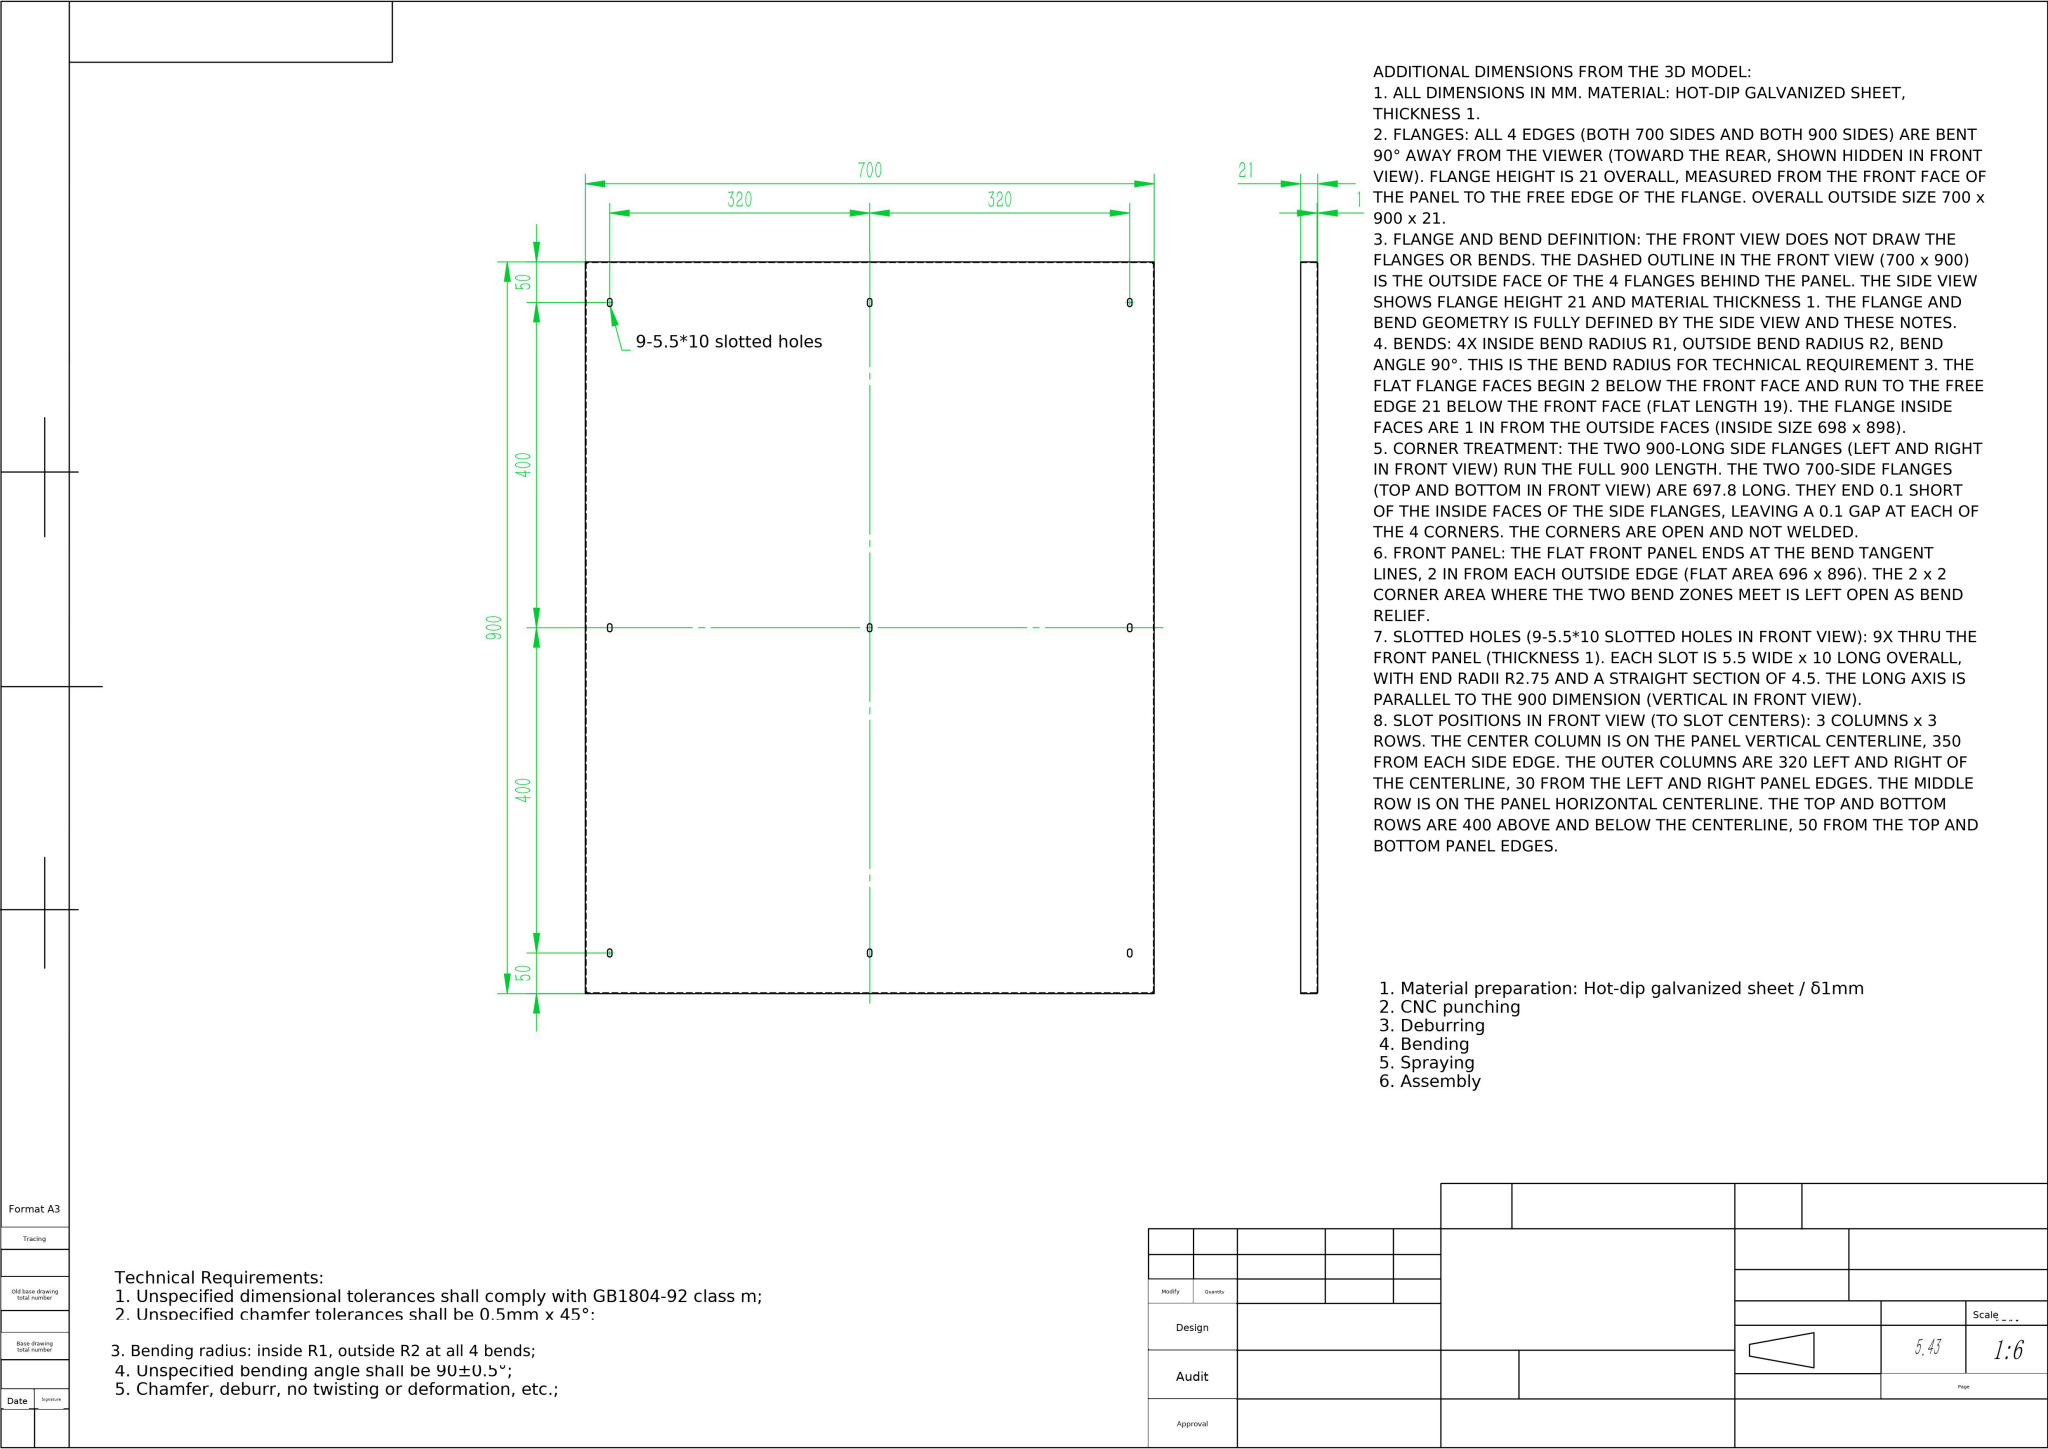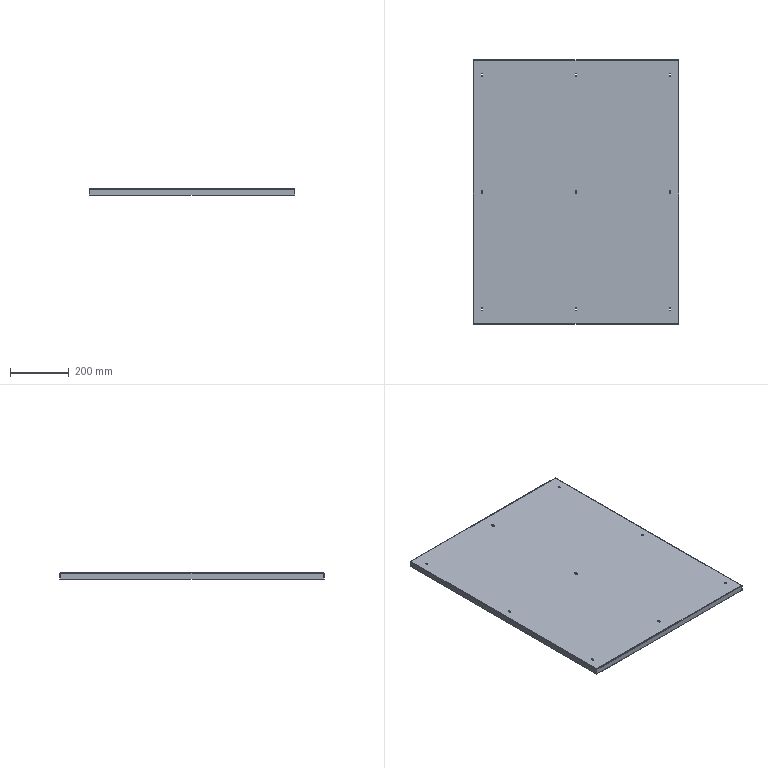Part | NX | mm | 1 solid | 74 faces | box 700 x 900 x 21 mm | volume 691412 mm3 | plane 40 | cylinder 26 | spline 8 | commonest cylinder face diameters 5.5 x18 2 x4 4 x4